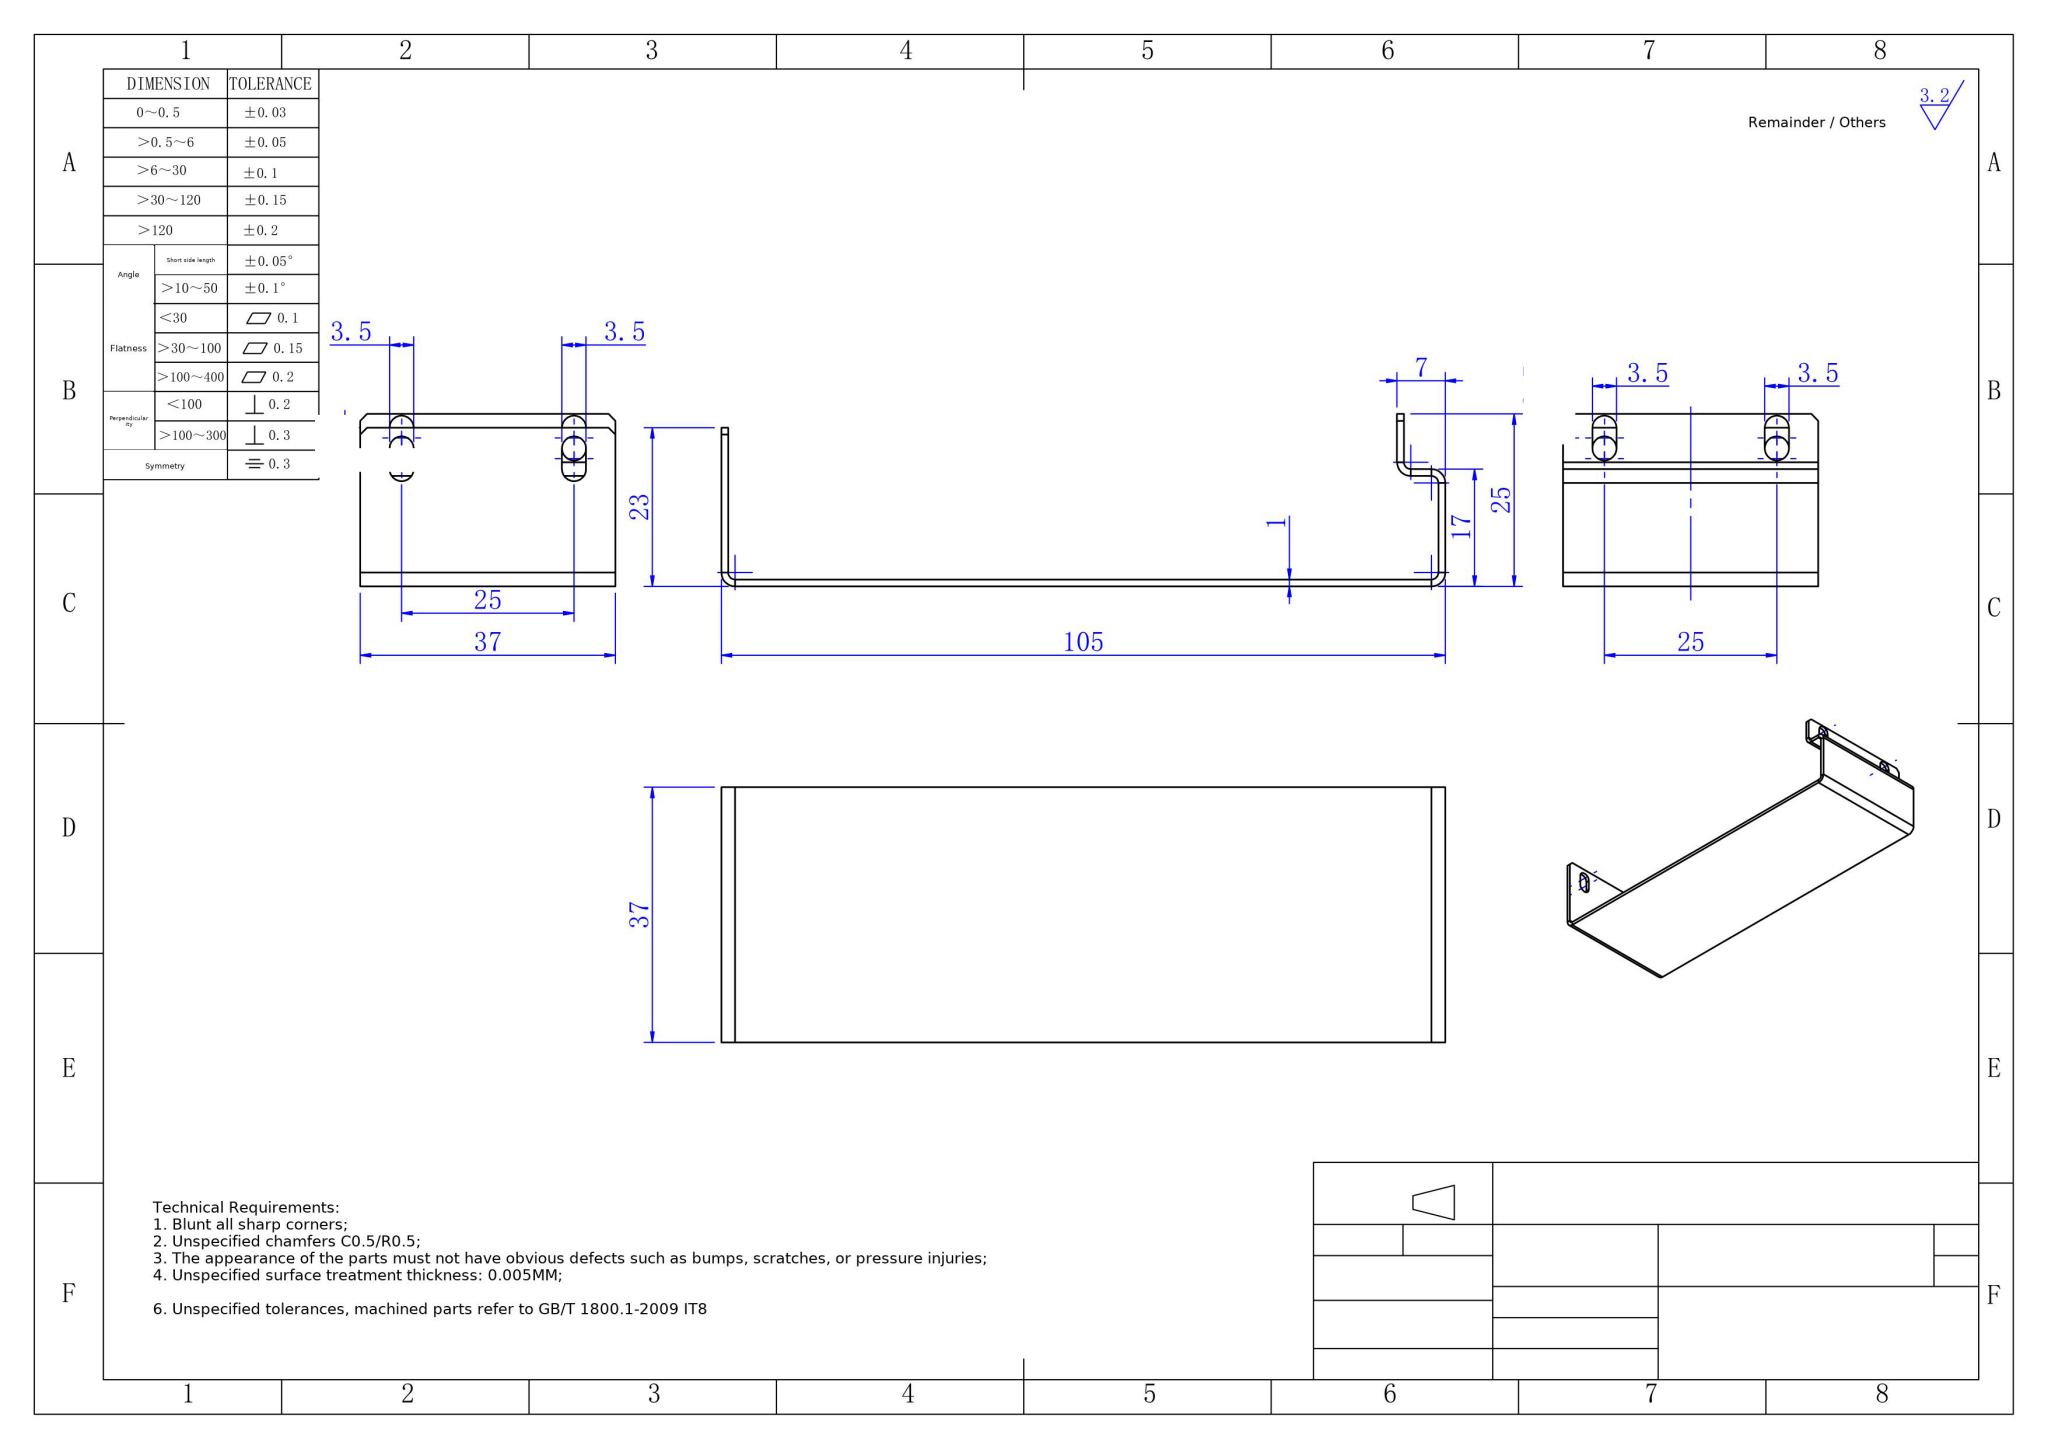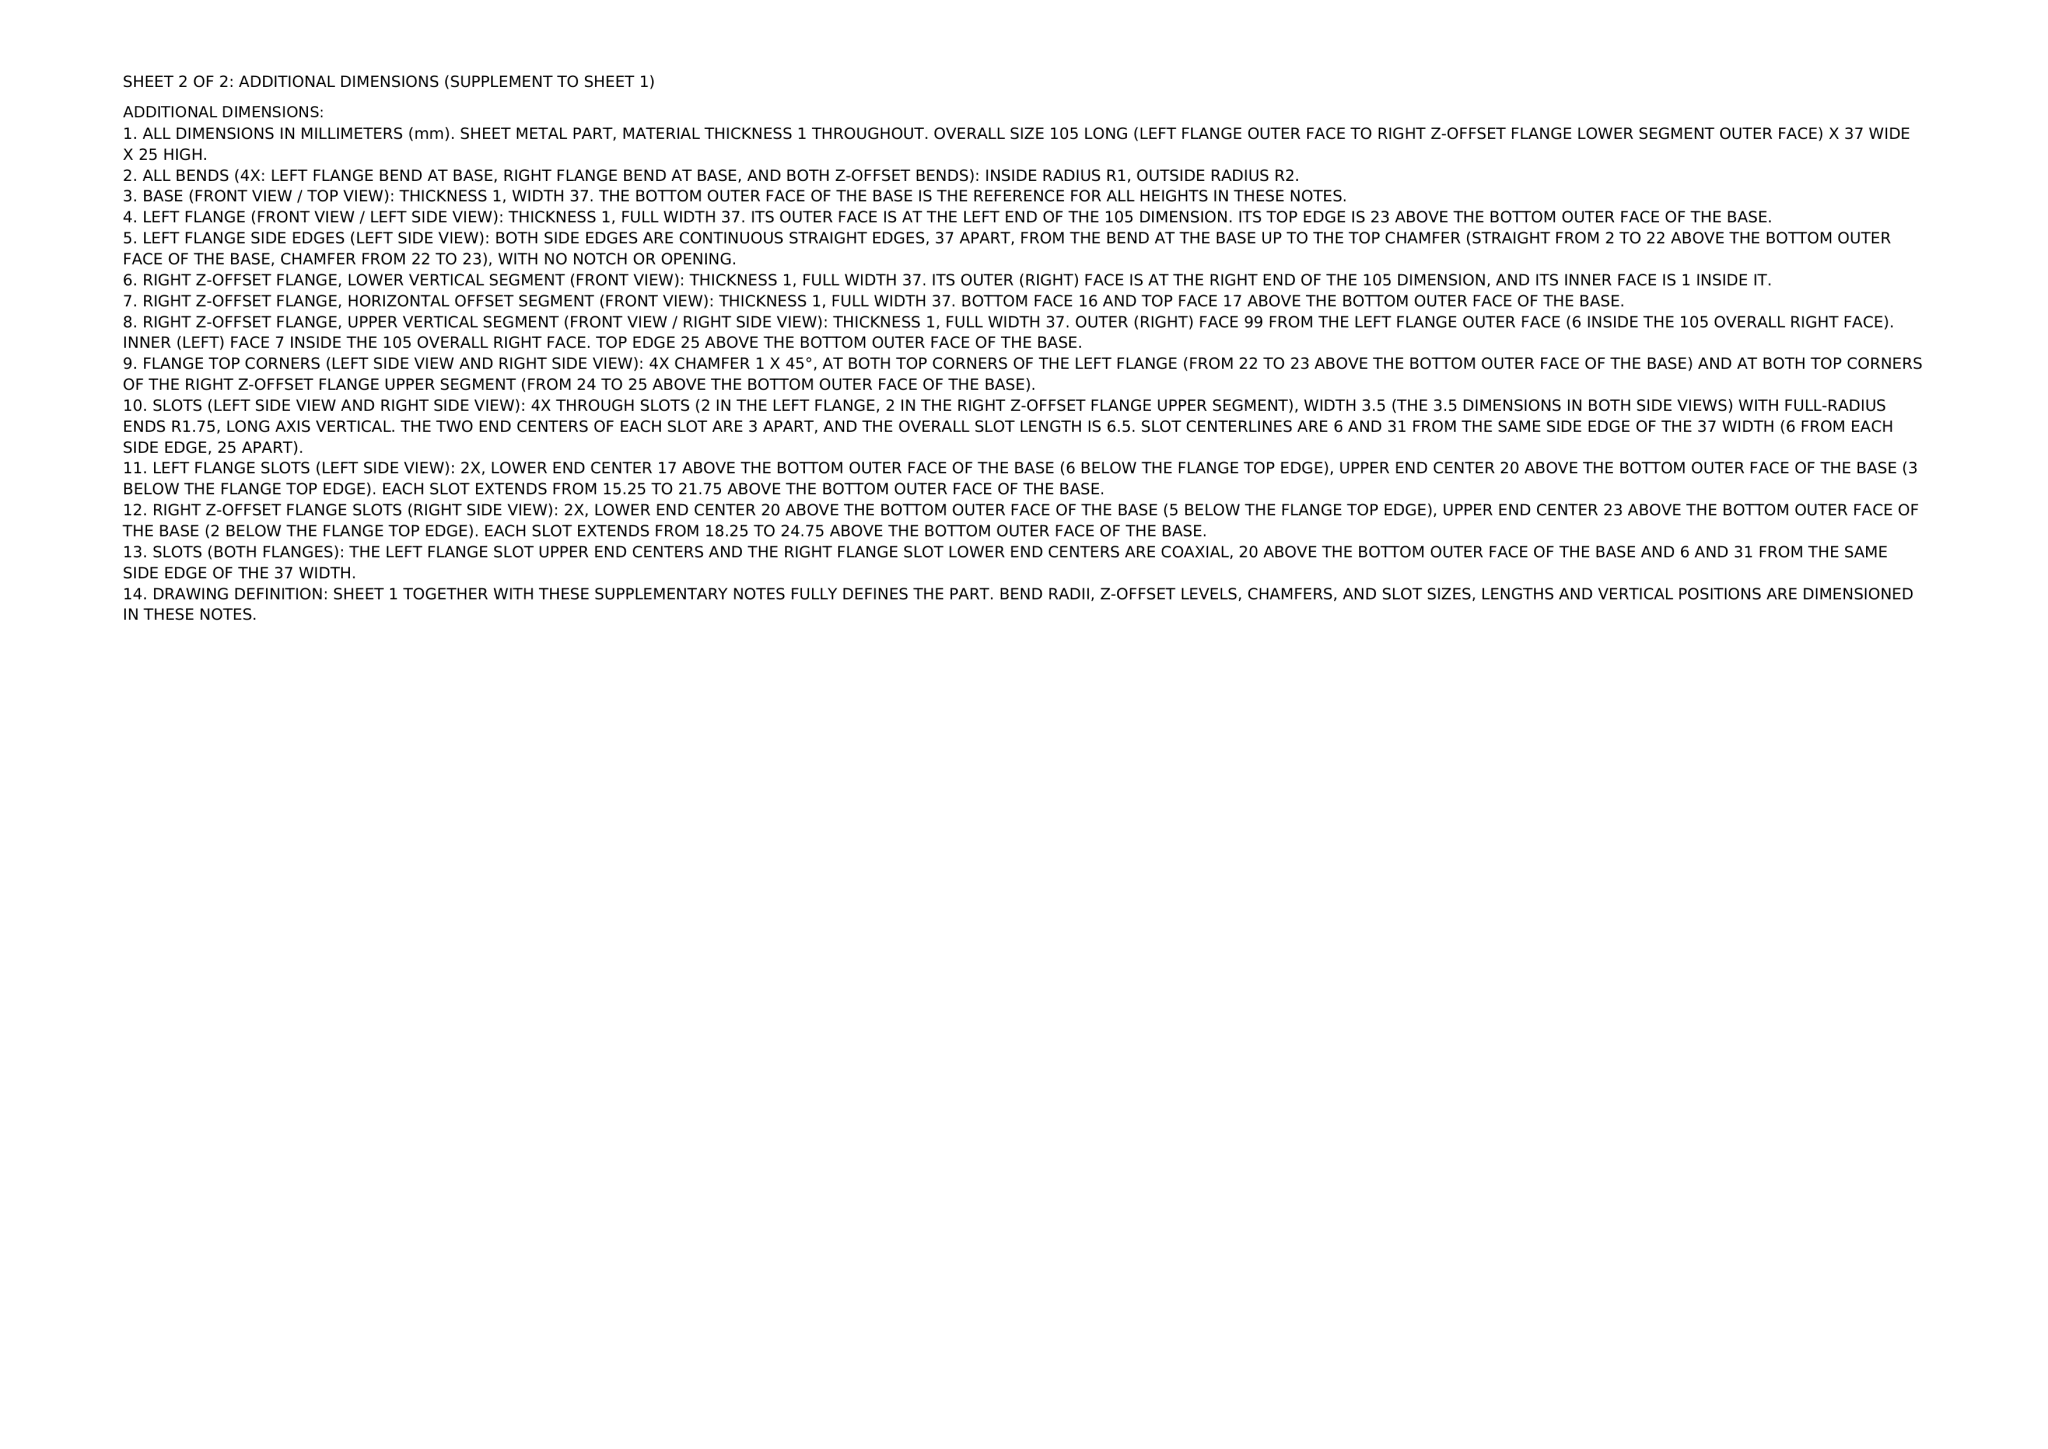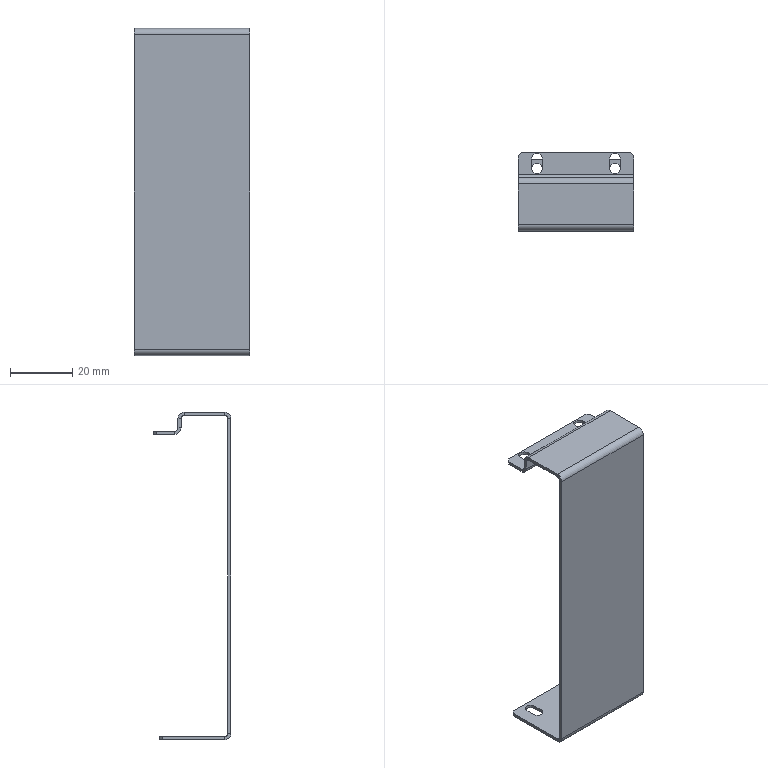Part | NX | mm | 1 solid | 58 faces | box 37 x 25 x 105 mm | volume 5631 mm3 | plane 42 | cylinder 16 | commonest cylinder face diameters 3.5 x8 4 x4 2 x4